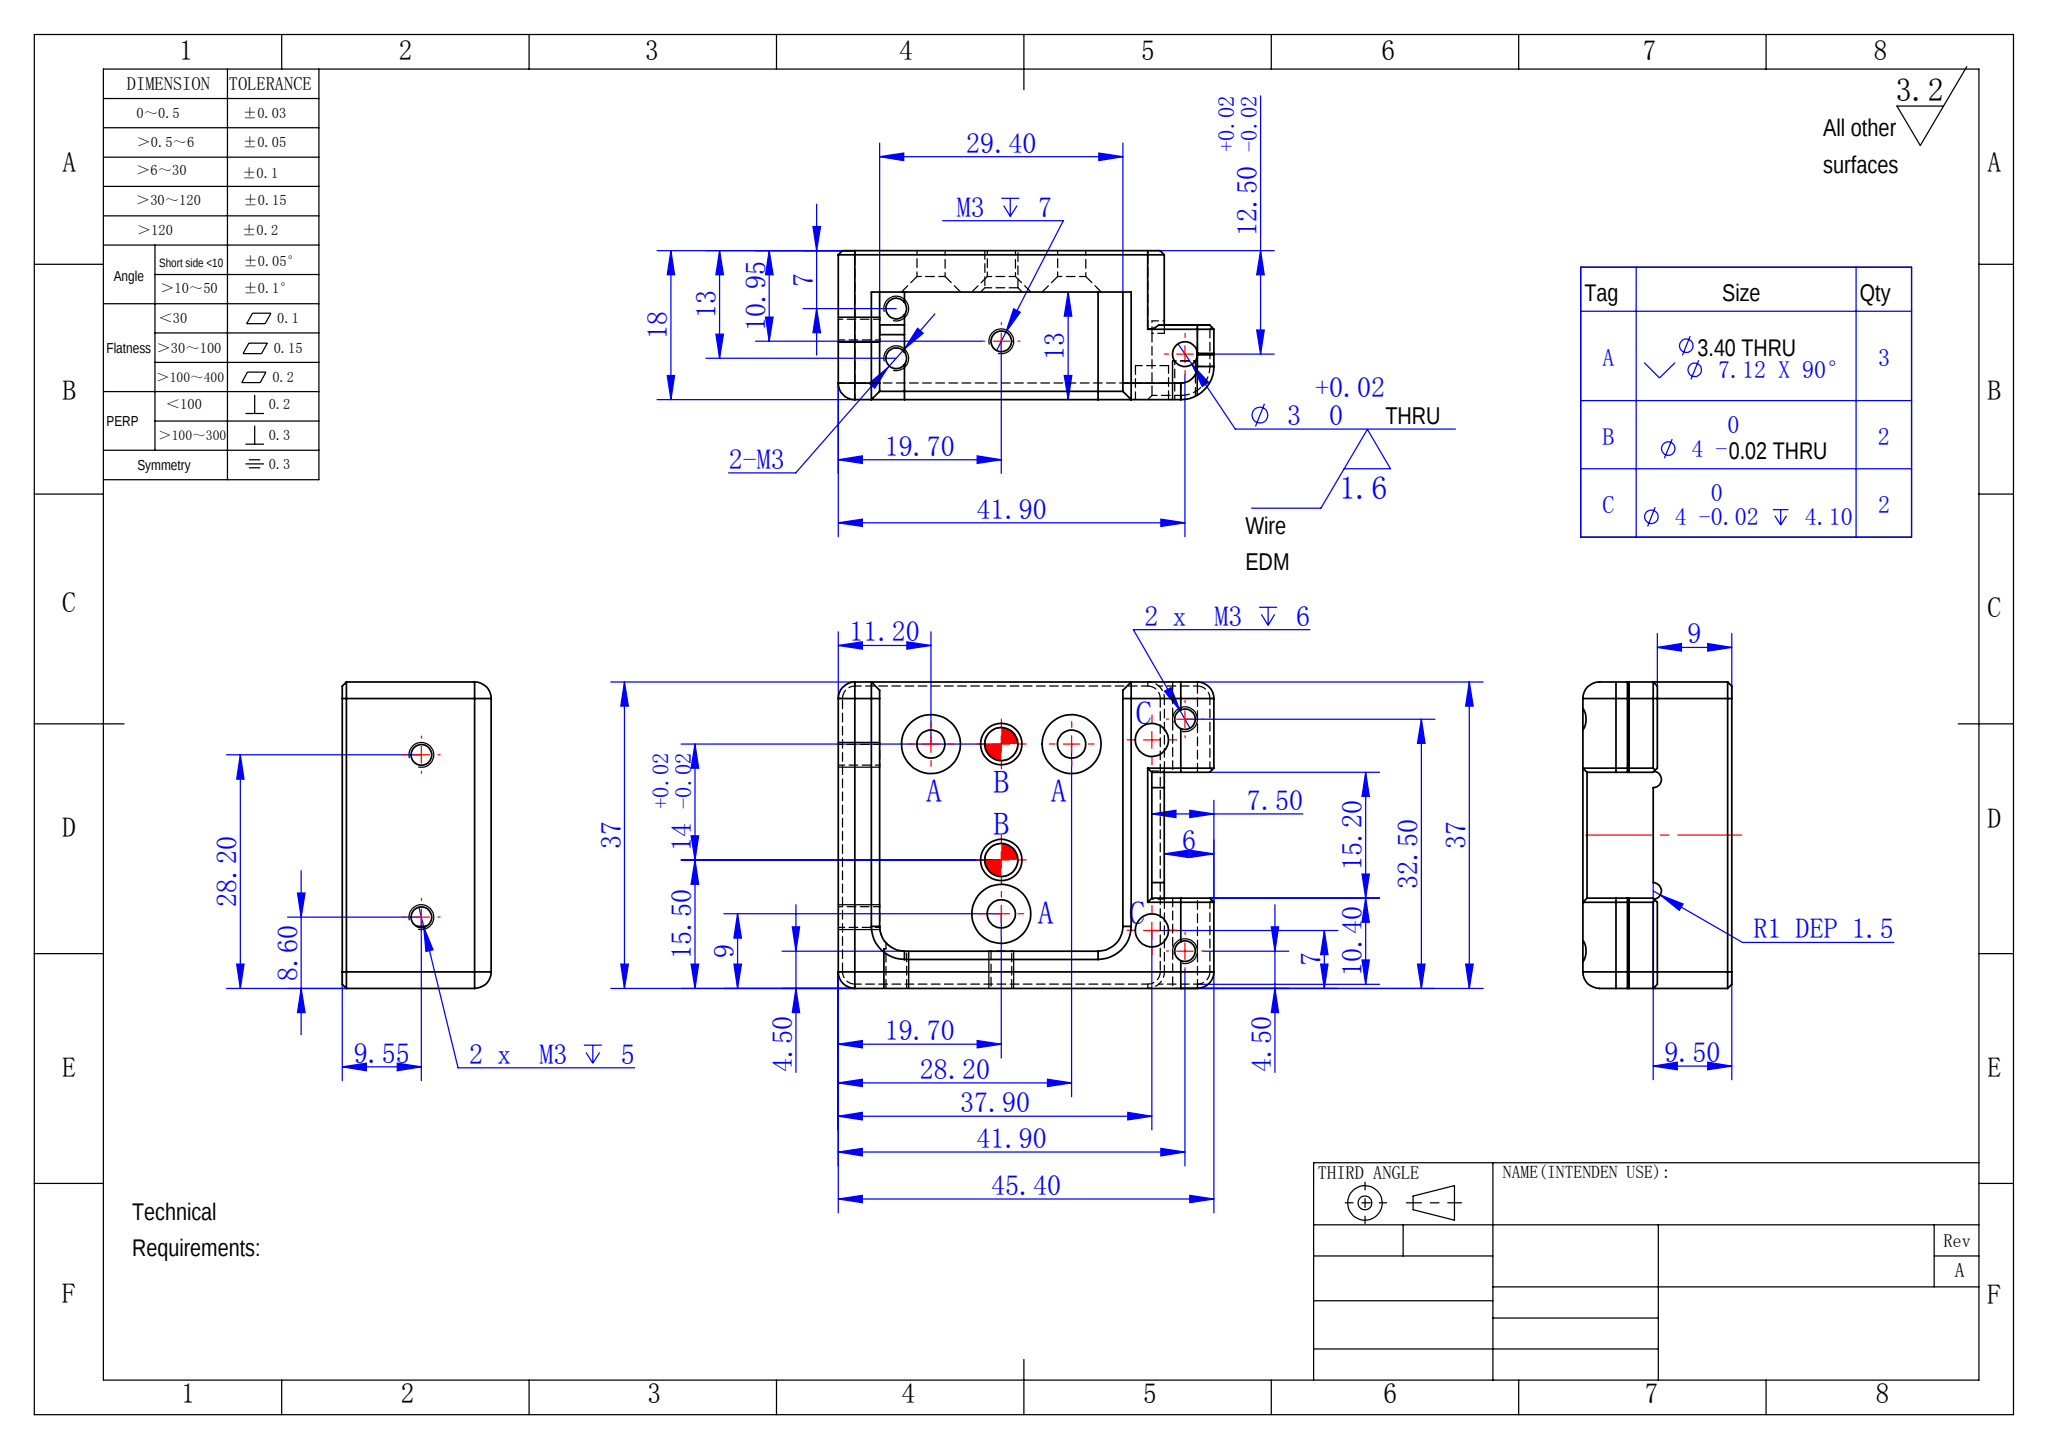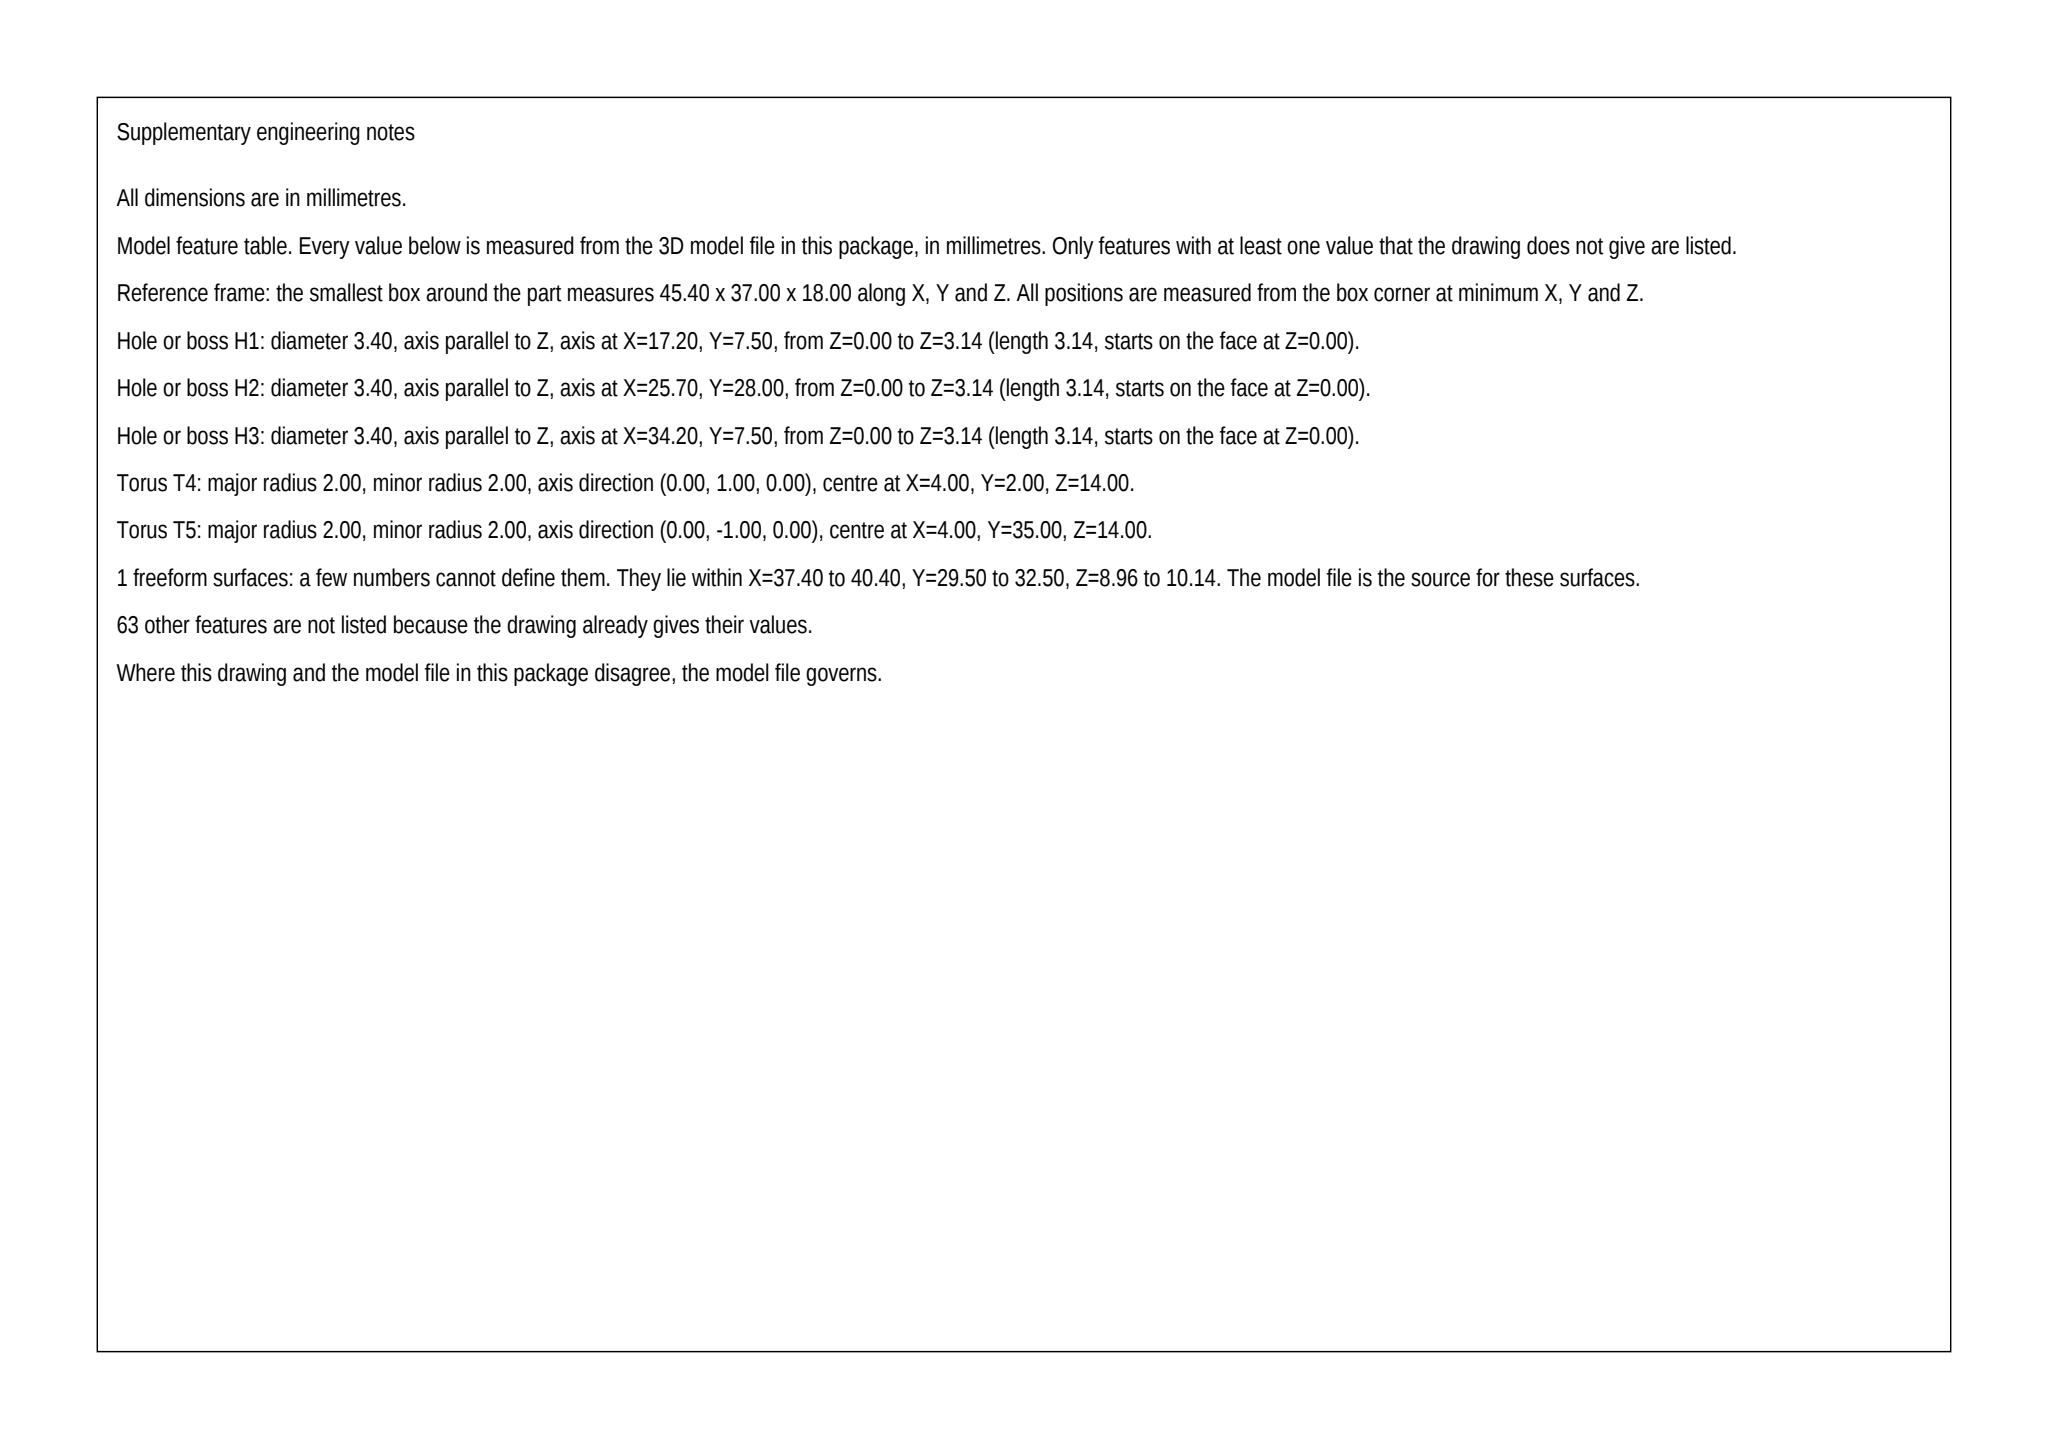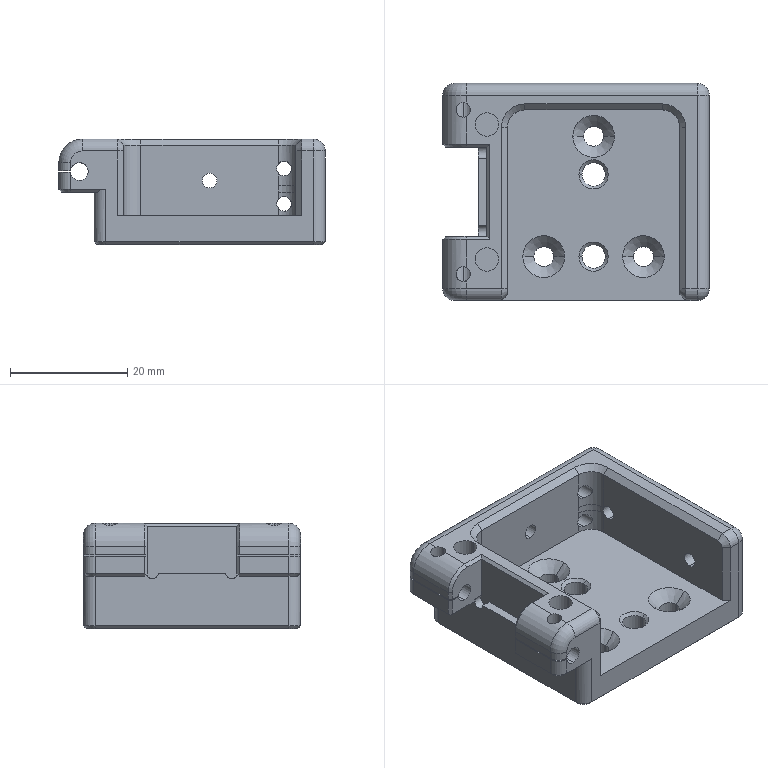Part | SolidWorks | mm | 1 solid | 130 faces | box 45.4 x 37 x 18 mm | volume 13781 mm3 | cylinder 53 | plane 50 | cone 22 | torus 2 | sphere 2 | spline 1 | commonest cylinder face diameters 4 x20 2.5 x14 3.4 x6 3 x6 6 x3 2 x2 8 x2